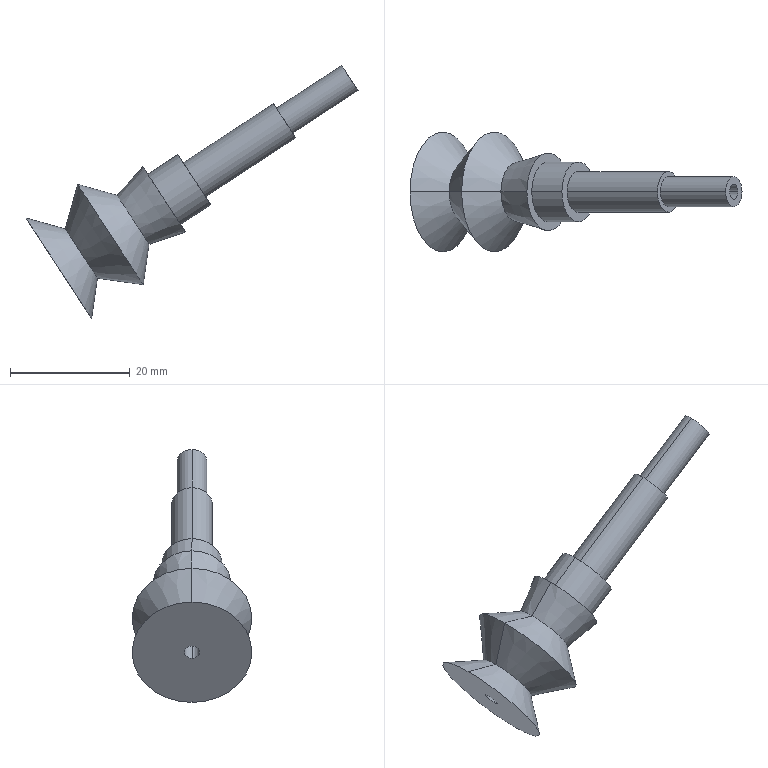Component | SolidWorks | NewSuctionCupGroup-1_SuctionCup1-1 | 1 solid | 21 faces | box 55.39 x 20 x 42.19 mm | volume 4409 mm3 | cylinder 8 | cone 8 | plane 5 | commonest cylinder face diameters 2.5 x2 10 x2 6.8 x2 5 x2
build123d program:
from build123d import *

# Parameters (mm, degrees)
SKETCH2_R          = 1.25
CUT_EXTRUDE1_DEPTH = 60.699


with BuildPart() as part:
    # Sketch1 → Revolve1 (revolve)
    with BuildSketch(Plane.XY, mode=Mode.PRIVATE) as revolve1_sk:
        Polygon((0, 0), (2.5, 0), (2.5, -13), (3.4, -13), (3.4, -31), (5, -31), (5, -37), (6.489, -37), (4.895, -43.22), (10, -47.704), (4.895, -53.516), (10, -58), (0, -58), align=None)
    revolve(revolve1_sk.sketch.rotate(Axis((0, 0, 0), (0, -1, 0)), 90), axis=Axis((0, 0, 0), (0, -1, 0)))

    # Sketch2 → Cut-Extrude1 (cut, through all)
    with BuildSketch(Plane.XZ.offset(58)):
        with Locations(Location((0, 0, 0), (0, 0, 270))):
            Circle(SKETCH2_R)
    extrude(amount=-CUT_EXTRUDE1_DEPTH, mode=Mode.SUBTRACT)


solid = part.part

# Placed as in the assembly
solid = solid.moved(Location((-65.517, -100.454, -13.641), (175.111, 33.07, -87.328)))
STEP:
#1=CARTESIAN_POINT('',(-2.606,-3.955,-0.4958));
#2=VERTEX_POINT('',#1);
#3=CARTESIAN_POINT('',(-2.552,-3.955,-0.5782));
#4=VERTEX_POINT('',#3);
#5=CARTESIAN_POINT('',(-2.579,-3.955,-0.537));
#6=DIRECTION('',(-0.8371,0.,-0.5471));
#7=DIRECTION('',(0.5471,0.,-0.8371));
#8=AXIS2_PLACEMENT_3D('',#5,#6,#7);
#9=CIRCLE('',#8,0.04921);
#10=EDGE_CURVE('',#2,#4,#9,.T.);
#11=ORIENTED_EDGE('',*,*,#10,.F.);
#12=CARTESIAN_POINT('',(-4.518,-3.955,-1.745));
#13=VERTEX_POINT('',#12);
#14=CARTESIAN_POINT('',(-2.606,-3.955,-0.4958));
#15=DIRECTION('',(-0.8371,0.,-0.5471));
#16=VECTOR('',#15,39.37);
#17=LINE('',#14,#16);
#18=EDGE_CURVE('',#2,#13,#17,.T.);
#19=ORIENTED_EDGE('',*,*,#18,.T.);
#20=CARTESIAN_POINT('',(-4.464,-3.955,-1.827));
#21=VERTEX_POINT('',#20);
#22=CARTESIAN_POINT('',(-4.491,-3.955,-1.786));
#23=DIRECTION('',(-0.8371,0.,-0.5471));
#24=DIRECTION('',(0.5471,0.,-0.8371));
#25=AXIS2_PLACEMENT_3D('',#22,#23,#24);
#26=CIRCLE('',#25,0.04921);
#27=EDGE_CURVE('',#13,#21,#26,.T.);
#28=ORIENTED_EDGE('',*,*,#27,.T.);
#29=CARTESIAN_POINT('',(-2.552,-3.955,-0.5782));
#30=DIRECTION('',(-0.8371,0.,-0.5471));
#31=VECTOR('',#30,39.37);
#32=LINE('',#29,#31);
#33=EDGE_CURVE('',#4,#21,#32,.T.);
#34=ORIENTED_EDGE('',*,*,#33,.F.);
#35=EDGE_LOOP('',(#11,#19,#28,#34));
#36=FACE_OUTER_BOUND('',#35,.T.);
#37=CARTESIAN_POINT('',(-2.579,-3.955,-0.537));
#38=DIRECTION('',(-0.8371,0.,-0.5471));
#39=DIRECTION('',(0.5471,0.,-0.8371));
#40=AXIS2_PLACEMENT_3D('',#37,#38,#39);
#41=CYLINDRICAL_SURFACE('',#40,0.04921);
#42=ADVANCED_FACE('',(#36),#41,.F.);
#43=CARTESIAN_POINT('',(-4.449,-3.955,-1.528));
#44=VERTEX_POINT('',#43);
#45=CARTESIAN_POINT('',(-4.238,-3.955,-1.851));
#46=VERTEX_POINT('',#45);
#47=CARTESIAN_POINT('',(-4.343,-3.955,-1.69));
#48=DIRECTION('',(0.8371,-0.,0.5471));
#49=DIRECTION('',(-0.5471,0.,0.8371));
#50=AXIS2_PLACEMENT_3D('',#47,#48,#49);
#51=CIRCLE('',#50,0.1927);
#52=EDGE_CURVE('',#44,#46,#51,.T.);
#53=ORIENTED_EDGE('',*,*,#52,.F.);
#54=CARTESIAN_POINT('',(-4.706,-3.955,-1.457));
#55=VERTEX_POINT('',#54);
#56=CARTESIAN_POINT('',(-4.706,-3.955,-1.457));
#57=DIRECTION('',(-0.9634,0.,0.2679));
#58=VECTOR('',#57,39.37);
#59=LINE('',#56,#58);
#60=EDGE_CURVE('',#44,#55,#59,.T.);
#61=ORIENTED_EDGE('',*,*,#60,.T.);
#62=CARTESIAN_POINT('',(-4.276,-3.955,-2.116));
#63=VERTEX_POINT('',#62);
#64=CARTESIAN_POINT('',(-4.491,-3.955,-1.786));
#65=DIRECTION('',(0.8371,-0.,0.5471));
#66=DIRECTION('',(-0.5471,0.,0.8371));
#67=AXIS2_PLACEMENT_3D('',#64,#65,#66);
#68=CIRCLE('',#67,0.3937);
#69=EDGE_CURVE('',#55,#63,#68,.T.);
#70=ORIENTED_EDGE('',*,*,#69,.T.);
#71=CARTESIAN_POINT('',(-4.276,-3.955,-2.116));
#72=DIRECTION('',(-0.1414,-0.,-0.99));
#73=VECTOR('',#72,39.37);
#74=LINE('',#71,#73);
#75=EDGE_CURVE('',#46,#63,#74,.T.);
#76=ORIENTED_EDGE('',*,*,#75,.F.);
#77=EDGE_LOOP('',(#53,#61,#70,#76));
#78=FACE_OUTER_BOUND('',#77,.T.);
#79=CARTESIAN_POINT('',(-4.491,-3.955,-1.786));
#80=DIRECTION('',(-0.8371,0.,-0.5471));
#81=DIRECTION('',(0.5471,-0.,-0.8371));
#82=AXIS2_PLACEMENT_3D('',#79,#80,#81);
#83=CONICAL_SURFACE('',#82,0.3937,0.8501);
#84=ADVANCED_FACE('',(#78),#83,.T.);
#85=ORIENTED_EDGE('',*,*,#52,.T.);
#86=CARTESIAN_POINT('',(-3.936,-3.955,-1.894));
#87=VERTEX_POINT('',#86);
#88=CARTESIAN_POINT('',(-4.238,-3.955,-1.851));
#89=DIRECTION('',(0.99,-0.,-0.1414));
#90=VECTOR('',#89,39.37);
#91=LINE('',#88,#90);
#92=EDGE_CURVE('',#46,#87,#91,.T.);
#93=ORIENTED_EDGE('',*,*,#92,.T.);
#94=CARTESIAN_POINT('',(-4.367,-3.955,-1.235));
#95=VERTEX_POINT('',#94);
#96=CARTESIAN_POINT('',(-4.152,-3.955,-1.564));
#97=DIRECTION('',(0.8371,-0.,0.5471));
#98=DIRECTION('',(-0.5471,0.,0.8371));
#99=AXIS2_PLACEMENT_3D('',#96,#97,#98);
#100=CIRCLE('',#99,0.3937);
#101=EDGE_CURVE('',#95,#87,#100,.T.);
#102=ORIENTED_EDGE('',*,*,#101,.F.);
#103=CARTESIAN_POINT('',(-4.449,-3.955,-1.528));
#104=DIRECTION('',(0.2679,0.,0.9634));
#105=VECTOR('',#104,39.37);
#106=LINE('',#103,#105);
#107=EDGE_CURVE('',#44,#95,#106,.T.);
#108=ORIENTED_EDGE('',*,*,#107,.F.);
#109=EDGE_LOOP('',(#85,#93,#102,#108));
#110=FACE_OUTER_BOUND('',#109,.T.);
#111=CARTESIAN_POINT('',(-4.343,-3.955,-1.69));
#112=DIRECTION('',(0.8371,-0.,0.5471));
#113=DIRECTION('',(-0.5471,0.,0.8371));
#114=AXIS2_PLACEMENT_3D('',#111,#112,#113);
#115=CONICAL_SURFACE('',#114,0.1927,0.7207);
#116=ADVANCED_FACE('',(#110),#115,.T.);
#117=CARTESIAN_POINT('',(-4.109,-3.955,-1.307));
#118=VERTEX_POINT('',#117);
#119=CARTESIAN_POINT('',(-3.898,-3.955,-1.629));
#120=VERTEX_POINT('',#119);
#121=CARTESIAN_POINT('',(-4.004,-3.955,-1.468));
#122=DIRECTION('',(0.8371,-0.,0.5471));
#123=DIRECTION('',(-0.5471,0.,0.8371));
#124=AXIS2_PLACEMENT_3D('',#121,#122,#123);
#125=CIRCLE('',#124,0.1927);
#126=EDGE_CURVE('',#118,#120,#125,.T.);
#127=ORIENTED_EDGE('',*,*,#126,.F.);
#128=CARTESIAN_POINT('',(-4.367,-3.955,-1.235));
#129=DIRECTION('',(-0.9634,0.,0.2679));
#130=VECTOR('',#129,39.37);
#131=LINE('',#128,#130);
#132=EDGE_CURVE('',#118,#95,#131,.T.);
#133=ORIENTED_EDGE('',*,*,#132,.T.);
#134=ORIENTED_EDGE('',*,*,#101,.T.);
#135=CARTESIAN_POINT('',(-3.936,-3.955,-1.894));
#136=DIRECTION('',(-0.1414,-0.,-0.99));
#137=VECTOR('',#136,39.37);
#138=LINE('',#135,#137);
#139=EDGE_CURVE('',#120,#87,#138,.T.);
#140=ORIENTED_EDGE('',*,*,#139,.F.);
#141=EDGE_LOOP('',(#127,#133,#134,#140));
#142=FACE_OUTER_BOUND('',#141,.T.);
#143=CARTESIAN_POINT('',(-4.152,-3.955,-1.564));
#144=DIRECTION('',(-0.8371,0.,-0.5471));
#145=DIRECTION('',(0.5471,-0.,-0.8371));
#146=AXIS2_PLACEMENT_3D('',#143,#144,#145);
#147=CONICAL_SURFACE('',#146,0.3937,0.8501);
#148=ADVANCED_FACE('',(#142),#147,.T.);
#149=ORIENTED_EDGE('',*,*,#126,.T.);
#150=CARTESIAN_POINT('',(-3.659,-3.955,-1.548));
#151=VERTEX_POINT('',#150);
#152=CARTESIAN_POINT('',(-3.898,-3.955,-1.629));
#153=DIRECTION('',(0.9467,-0.,0.3221));
#154=VECTOR('',#153,39.37);
#155=LINE('',#152,#154);
#156=EDGE_CURVE('',#120,#151,#155,.T.);
#157=ORIENTED_EDGE('',*,*,#156,.T.);
#158=CARTESIAN_POINT('',(-3.939,-3.955,-1.12));
#159=VERTEX_POINT('',#158);
#160=CARTESIAN_POINT('',(-3.799,-3.955,-1.334));
#161=DIRECTION('',(0.8371,-0.,0.5471));
#162=DIRECTION('',(-0.5471,0.,0.8371));
#163=AXIS2_PLACEMENT_3D('',#160,#161,#162);
#164=CIRCLE('',#163,0.2555);
#165=EDGE_CURVE('',#159,#151,#164,.T.);
#166=ORIENTED_EDGE('',*,*,#165,.F.);
#167=CARTESIAN_POINT('',(-4.109,-3.955,-1.307));
#168=DIRECTION('',(0.6751,-0.,0.7377));
#169=VECTOR('',#168,39.37);
#170=LINE('',#167,#169);
#171=EDGE_CURVE('',#118,#159,#170,.T.);
#172=ORIENTED_EDGE('',*,*,#171,.F.);
#173=EDGE_LOOP('',(#149,#157,#166,#172));
#174=FACE_OUTER_BOUND('',#173,.T.);
#175=CARTESIAN_POINT('',(-4.004,-3.955,-1.468));
#176=DIRECTION('',(0.8371,-0.,0.5471));
#177=DIRECTION('',(-0.5471,0.,0.8371));
#178=AXIS2_PLACEMENT_3D('',#175,#176,#177);
#179=CONICAL_SURFACE('',#178,0.1927,0.2509);
#180=ADVANCED_FACE('',(#174),#179,.T.);
#181=CARTESIAN_POINT('',(-3.906,-3.955,-1.169));
#182=VERTEX_POINT('',#181);
#183=CARTESIAN_POINT('',(-3.691,-3.955,-1.499));
#184=VERTEX_POINT('',#183);
#185=CARTESIAN_POINT('',(-3.799,-3.955,-1.334));
#186=DIRECTION('',(0.8371,-0.,0.5471));
#187=DIRECTION('',(-0.5471,0.,0.8371));
#188=AXIS2_PLACEMENT_3D('',#185,#186,#187);
#189=CIRCLE('',#188,0.1969);
#190=EDGE_CURVE('',#182,#184,#189,.T.);
#191=ORIENTED_EDGE('',*,*,#190,.T.);
#192=CARTESIAN_POINT('',(-3.493,-3.955,-1.369));
#193=VERTEX_POINT('',#192);
#194=CARTESIAN_POINT('',(-2.472,-3.955,-0.7018));
#195=DIRECTION('',(0.8371,-0.,0.5471));
#196=VECTOR('',#195,39.37);
#197=LINE('',#194,#196);
#198=EDGE_CURVE('',#184,#193,#197,.T.);
#199=ORIENTED_EDGE('',*,*,#198,.T.);
#200=CARTESIAN_POINT('',(-3.709,-3.955,-1.04));
#201=VERTEX_POINT('',#200);
#202=CARTESIAN_POINT('',(-3.601,-3.955,-1.205));
#203=DIRECTION('',(0.8371,-0.,0.5471));
#204=DIRECTION('',(-0.5471,0.,0.8371));
#205=AXIS2_PLACEMENT_3D('',#202,#203,#204);
#206=CIRCLE('',#205,0.1969);
#207=EDGE_CURVE('',#201,#193,#206,.T.);
#208=ORIENTED_EDGE('',*,*,#207,.F.);
#209=CARTESIAN_POINT('',(-2.687,-3.955,-0.3723));
#210=DIRECTION('',(0.8371,-0.,0.5471));
#211=VECTOR('',#210,39.37);
#212=LINE('',#209,#211);
#213=EDGE_CURVE('',#182,#201,#212,.T.);
#214=ORIENTED_EDGE('',*,*,#213,.F.);
#215=EDGE_LOOP('',(#191,#199,#208,#214));
#216=FACE_OUTER_BOUND('',#215,.T.);
#217=CARTESIAN_POINT('',(-2.579,-3.955,-0.537));
#218=DIRECTION('',(0.8371,-0.,0.5471));
#219=DIRECTION('',(-0.5471,0.,0.8371));
#220=AXIS2_PLACEMENT_3D('',#217,#218,#219);
#221=CYLINDRICAL_SURFACE('',#220,0.1969);
#222=ADVANCED_FACE('',(#216),#221,.T.);
#223=CARTESIAN_POINT('',(-3.674,-3.955,-1.093));
#224=VERTEX_POINT('',#223);
#225=CARTESIAN_POINT('',(-3.528,-3.955,-1.317));
#226=VERTEX_POINT('',#225);
#227=CARTESIAN_POINT('',(-3.601,-3.955,-1.205));
#228=DIRECTION('',(0.8371,-0.,0.5471));
#229=DIRECTION('',(-0.5471,0.,0.8371));
#230=AXIS2_PLACEMENT_3D('',#227,#228,#229);
#231=CIRCLE('',#230,0.1339);
#232=EDGE_CURVE('',#224,#226,#231,.T.);
#233=ORIENTED_EDGE('',*,*,#232,.T.);
#234=CARTESIAN_POINT('',(-2.935,-3.955,-0.9291));
#235=VERTEX_POINT('',#234);
#236=CARTESIAN_POINT('',(-2.506,-3.955,-0.6491));
#237=DIRECTION('',(0.8371,-0.,0.5471));
#238=VECTOR('',#237,39.37);
#239=LINE('',#236,#238);
#240=EDGE_CURVE('',#226,#235,#239,.T.);
#241=ORIENTED_EDGE('',*,*,#240,.T.);
#242=CARTESIAN_POINT('',(-3.081,-3.955,-0.705));
#243=VERTEX_POINT('',#242);
#244=CARTESIAN_POINT('',(-3.008,-3.955,-0.817));
#245=DIRECTION('',(0.8371,-0.,0.5471));
#246=DIRECTION('',(-0.5471,0.,0.8371));
#247=AXIS2_PLACEMENT_3D('',#244,#245,#246);
#248=CIRCLE('',#247,0.1339);
#249=EDGE_CURVE('',#243,#235,#248,.T.);
#250=ORIENTED_EDGE('',*,*,#249,.F.);
#251=CARTESIAN_POINT('',(-2.653,-3.955,-0.425));
#252=DIRECTION('',(0.8371,-0.,0.5471));
#253=VECTOR('',#252,39.37);
#254=LINE('',#251,#253);
#255=EDGE_CURVE('',#224,#243,#254,.T.);
#256=ORIENTED_EDGE('',*,*,#255,.F.);
#257=EDGE_LOOP('',(#233,#241,#250,#256));
#258=FACE_OUTER_BOUND('',#257,.T.);
#259=CARTESIAN_POINT('',(-2.579,-3.955,-0.537));
#260=DIRECTION('',(0.8371,-0.,0.5471));
#261=DIRECTION('',(-0.5471,0.,0.8371));
#262=AXIS2_PLACEMENT_3D('',#259,#260,#261);
#263=CYLINDRICAL_SURFACE('',#262,0.1339);
#264=ADVANCED_FACE('',(#258),#263,.T.);
#265=CARTESIAN_POINT('',(-3.062,-3.955,-0.7346));
#266=VERTEX_POINT('',#265);
#267=CARTESIAN_POINT('',(-2.954,-3.955,-0.8994));
#268=VERTEX_POINT('',#267);
#269=CARTESIAN_POINT('',(-3.008,-3.955,-0.817));
#270=DIRECTION('',(0.8371,-0.,0.5471));
#271=DIRECTION('',(-0.5471,0.,0.8371));
#272=AXIS2_PLACEMENT_3D('',#269,#270,#271);
#273=CIRCLE('',#272,0.09843);
#274=EDGE_CURVE('',#266,#268,#273,.T.);
#275=ORIENTED_EDGE('',*,*,#274,.T.);
#276=CARTESIAN_POINT('',(-2.526,-3.955,-0.6194));
#277=VERTEX_POINT('',#276);
#278=CARTESIAN_POINT('',(-2.526,-3.955,-0.6194));
#279=DIRECTION('',(0.8371,-0.,0.5471));
#280=VECTOR('',#279,39.37);
#281=LINE('',#278,#280);
#282=EDGE_CURVE('',#268,#277,#281,.T.);
#283=ORIENTED_EDGE('',*,*,#282,.T.);
#284=CARTESIAN_POINT('',(-2.633,-3.955,-0.4546));
#285=VERTEX_POINT('',#284);
#286=CARTESIAN_POINT('',(-2.579,-3.955,-0.537));
#287=DIRECTION('',(0.8371,-0.,0.5471));
#288=DIRECTION('',(-0.5471,0.,0.8371));
#289=AXIS2_PLACEMENT_3D('',#286,#287,#288);
#290=CIRCLE('',#289,0.09843);
#291=EDGE_CURVE('',#285,#277,#290,.T.);
#292=ORIENTED_EDGE('',*,*,#291,.F.);
#293=CARTESIAN_POINT('',(-2.633,-3.955,-0.4546));
#294=DIRECTION('',(0.8371,-0.,0.5471));
#295=VECTOR('',#294,39.37);
#296=LINE('',#293,#295);
#297=EDGE_CURVE('',#266,#285,#296,.T.);
#298=ORIENTED_EDGE('',*,*,#297,.F.);
#299=EDGE_LOOP('',(#275,#283,#292,#298));
#300=FACE_OUTER_BOUND('',#299,.T.);
#301=CARTESIAN_POINT('',(-2.579,-3.955,-0.537));
#302=DIRECTION('',(0.8371,-0.,0.5471));
#303=DIRECTION('',(-0.5471,0.,0.8371));
#304=AXIS2_PLACEMENT_3D('',#301,#302,#303);
#305=CYLINDRICAL_SURFACE('',#304,0.09843);
#306=ADVANCED_FACE('',(#300),#305,.T.);
#307=CARTESIAN_POINT('',(-2.579,-3.955,-0.537));
#308=DIRECTION('',(-0.8371,0.,-0.5471));
#309=DIRECTION('',(0.5471,0.,-0.8371));
#310=AXIS2_PLACEMENT_3D('',#307,#308,#309);
#311=CIRCLE('',#310,0.04921);
#312=EDGE_CURVE('',#4,#2,#311,.T.);
#313=ORIENTED_EDGE('',*,*,#312,.T.);
#314=ORIENTED_EDGE('',*,*,#10,.T.);
#315=EDGE_LOOP('',(#313,#314));
#316=FACE_BOUND('',#315,.T.);
#317=ORIENTED_EDGE('',*,*,#291,.T.);
#318=CARTESIAN_POINT('',(-2.579,-3.955,-0.537));
#319=DIRECTION('',(0.8371,-0.,0.5471));
#320=DIRECTION('',(-0.5471,0.,0.8371));
#321=AXIS2_PLACEMENT_3D('',#318,#319,#320);
#322=CIRCLE('',#321,0.09843);
#323=EDGE_CURVE('',#277,#285,#322,.T.);
#324=ORIENTED_EDGE('',*,*,#323,.T.);
#325=EDGE_LOOP('',(#317,#324));
#326=FACE_OUTER_BOUND('',#325,.T.);
#327=CARTESIAN_POINT('',(-2.579,-3.955,-0.537));
#328=DIRECTION('',(-0.8371,0.,-0.5471));
#329=DIRECTION('',(0.5471,-0.,-0.8371));
#330=AXIS2_PLACEMENT_3D('',#327,#328,#329);
#331=PLANE('',#330);
#332=ADVANCED_FACE('',(#316,#326),#331,.F.);
#333=ORIENTED_EDGE('',*,*,#282,.F.);
#334=CARTESIAN_POINT('',(-3.008,-3.955,-0.817));
#335=DIRECTION('',(0.8371,-0.,0.5471));
#336=DIRECTION('',(-0.5471,0.,0.8371));
#337=AXIS2_PLACEMENT_3D('',#334,#335,#336);
#338=CIRCLE('',#337,0.09843);
#339=EDGE_CURVE('',#268,#266,#338,.T.);
#340=ORIENTED_EDGE('',*,*,#339,.T.);
#341=ORIENTED_EDGE('',*,*,#297,.T.);
#342=ORIENTED_EDGE('',*,*,#323,.F.);
#343=EDGE_LOOP('',(#333,#340,#341,#342));
#344=FACE_OUTER_BOUND('',#343,.T.);
#345=CARTESIAN_POINT('',(-2.579,-3.955,-0.537));
#346=DIRECTION('',(0.8371,-0.,0.5471));
#347=DIRECTION('',(-0.5471,0.,0.8371));
#348=AXIS2_PLACEMENT_3D('',#345,#346,#347);
#349=CYLINDRICAL_SURFACE('',#348,0.09843);
#350=ADVANCED_FACE('',(#344),#349,.T.);
#351=ORIENTED_EDGE('',*,*,#274,.F.);
#352=ORIENTED_EDGE('',*,*,#339,.F.);
#353=EDGE_LOOP('',(#351,#352));
#354=FACE_BOUND('',#353,.T.);
#355=ORIENTED_EDGE('',*,*,#249,.T.);
#356=CARTESIAN_POINT('',(-3.008,-3.955,-0.817));
#357=DIRECTION('',(0.8371,-0.,0.5471));
#358=DIRECTION('',(-0.5471,0.,0.8371));
#359=AXIS2_PLACEMENT_3D('',#356,#357,#358);
#360=CIRCLE('',#359,0.1339);
#361=EDGE_CURVE('',#235,#243,#360,.T.);
#362=ORIENTED_EDGE('',*,*,#361,.T.);
#363=EDGE_LOOP('',(#355,#362));
#364=FACE_OUTER_BOUND('',#363,.T.);
#365=CARTESIAN_POINT('',(-3.008,-4.053,-0.817));
#366=DIRECTION('',(-0.8371,0.,-0.5471));
#367=DIRECTION('',(0.5471,-0.,-0.8371));
#368=AXIS2_PLACEMENT_3D('',#365,#366,#367);
#369=PLANE('',#368);
#370=ADVANCED_FACE('',(#354,#364),#369,.F.);
#371=ORIENTED_EDGE('',*,*,#240,.F.);
#372=CARTESIAN_POINT('',(-3.601,-3.955,-1.205));
#373=DIRECTION('',(0.8371,-0.,0.5471));
#374=DIRECTION('',(-0.5471,0.,0.8371));
#375=AXIS2_PLACEMENT_3D('',#372,#373,#374);
#376=CIRCLE('',#375,0.1339);
#377=EDGE_CURVE('',#226,#224,#376,.T.);
#378=ORIENTED_EDGE('',*,*,#377,.T.);
#379=ORIENTED_EDGE('',*,*,#255,.T.);
#380=ORIENTED_EDGE('',*,*,#361,.F.);
#381=EDGE_LOOP('',(#371,#378,#379,#380));
#382=FACE_OUTER_BOUND('',#381,.T.);
#383=CARTESIAN_POINT('',(-2.579,-3.955,-0.537));
#384=DIRECTION('',(0.8371,-0.,0.5471));
#385=DIRECTION('',(-0.5471,0.,0.8371));
#386=AXIS2_PLACEMENT_3D('',#383,#384,#385);
#387=CYLINDRICAL_SURFACE('',#386,0.1339);
#388=ADVANCED_FACE('',(#382),#387,.T.);
#389=ORIENTED_EDGE('',*,*,#232,.F.);
#390=ORIENTED_EDGE('',*,*,#377,.F.);
#391=EDGE_LOOP('',(#389,#390));
#392=FACE_BOUND('',#391,.T.);
#393=ORIENTED_EDGE('',*,*,#207,.T.);
#394=CARTESIAN_POINT('',(-3.601,-3.955,-1.205));
#395=DIRECTION('',(0.8371,-0.,0.5471));
#396=DIRECTION('',(-0.5471,0.,0.8371));
#397=AXIS2_PLACEMENT_3D('',#394,#395,#396);
#398=CIRCLE('',#397,0.1969);
#399=EDGE_CURVE('',#193,#201,#398,.T.);
#400=ORIENTED_EDGE('',*,*,#399,.T.);
#401=EDGE_LOOP('',(#393,#400));
#402=FACE_OUTER_BOUND('',#401,.T.);
#403=CARTESIAN_POINT('',(-3.601,-4.089,-1.205));
#404=DIRECTION('',(-0.8371,0.,-0.5471));
#405=DIRECTION('',(0.5471,-0.,-0.8371));
#406=AXIS2_PLACEMENT_3D('',#403,#404,#405);
#407=PLANE('',#406);
#408=ADVANCED_FACE('',(#392,#402),#407,.F.);
#409=ORIENTED_EDGE('',*,*,#198,.F.);
#410=CARTESIAN_POINT('',(-3.799,-3.955,-1.334));
#411=DIRECTION('',(0.8371,-0.,0.5471));
#412=DIRECTION('',(-0.5471,0.,0.8371));
#413=AXIS2_PLACEMENT_3D('',#410,#411,#412);
#414=CIRCLE('',#413,0.1969);
#415=EDGE_CURVE('',#184,#182,#414,.T.);
#416=ORIENTED_EDGE('',*,*,#415,.T.);
#417=ORIENTED_EDGE('',*,*,#213,.T.);
#418=ORIENTED_EDGE('',*,*,#399,.F.);
#419=EDGE_LOOP('',(#409,#416,#417,#418));
#420=FACE_OUTER_BOUND('',#419,.T.);
#421=CARTESIAN_POINT('',(-2.579,-3.955,-0.537));
#422=DIRECTION('',(0.8371,-0.,0.5471));
#423=DIRECTION('',(-0.5471,0.,0.8371));
#424=AXIS2_PLACEMENT_3D('',#421,#422,#423);
#425=CYLINDRICAL_SURFACE('',#424,0.1969);
#426=ADVANCED_FACE('',(#420),#425,.T.);
#427=ORIENTED_EDGE('',*,*,#190,.F.);
#428=ORIENTED_EDGE('',*,*,#415,.F.);
#429=EDGE_LOOP('',(#427,#428));
#430=FACE_BOUND('',#429,.T.);
#431=ORIENTED_EDGE('',*,*,#165,.T.);
#432=CARTESIAN_POINT('',(-3.799,-3.955,-1.334));
#433=DIRECTION('',(0.8371,-0.,0.5471));
#434=DIRECTION('',(-0.5471,0.,0.8371));
#435=AXIS2_PLACEMENT_3D('',#432,#433,#434);
#436=CIRCLE('',#435,0.2555);
#437=EDGE_CURVE('',#151,#159,#436,.T.);
#438=ORIENTED_EDGE('',*,*,#437,.T.);
#439=EDGE_LOOP('',(#431,#438));
#440=FACE_OUTER_BOUND('',#439,.T.);
#441=CARTESIAN_POINT('',(-3.799,-4.152,-1.334));
#442=DIRECTION('',(-0.8371,0.,-0.5471));
#443=DIRECTION('',(0.5471,-0.,-0.8371));
#444=AXIS2_PLACEMENT_3D('',#441,#442,#443);
#445=PLANE('',#444);
#446=ADVANCED_FACE('',(#430,#440),#445,.F.);
#447=ORIENTED_EDGE('',*,*,#156,.F.);
#448=CARTESIAN_POINT('',(-4.004,-3.955,-1.468));
#449=DIRECTION('',(0.8371,-0.,0.5471));
#450=DIRECTION('',(-0.5471,0.,0.8371));
#451=AXIS2_PLACEMENT_3D('',#448,#449,#450);
#452=CIRCLE('',#451,0.1927);
#453=EDGE_CURVE('',#120,#118,#452,.T.);
#454=ORIENTED_EDGE('',*,*,#453,.T.);
#455=ORIENTED_EDGE('',*,*,#171,.T.);
#456=ORIENTED_EDGE('',*,*,#437,.F.);
#457=EDGE_LOOP('',(#447,#454,#455,#456));
#458=FACE_OUTER_BOUND('',#457,.T.);
#459=CARTESIAN_POINT('',(-4.004,-3.955,-1.468));
#460=DIRECTION('',(0.8371,-0.,0.5471));
#461=DIRECTION('',(-0.5471,0.,0.8371));
#462=AXIS2_PLACEMENT_3D('',#459,#460,#461);
#463=CONICAL_SURFACE('',#462,0.1927,0.2509);
#464=ADVANCED_FACE('',(#458),#463,.T.);
#465=ORIENTED_EDGE('',*,*,#132,.F.);
#466=ORIENTED_EDGE('',*,*,#453,.F.);
#467=ORIENTED_EDGE('',*,*,#139,.T.);
#468=CARTESIAN_POINT('',(-4.152,-3.955,-1.564));
#469=DIRECTION('',(0.8371,-0.,0.5471));
#470=DIRECTION('',(-0.5471,0.,0.8371));
#471=AXIS2_PLACEMENT_3D('',#468,#469,#470);
#472=CIRCLE('',#471,0.3937);
#473=EDGE_CURVE('',#87,#95,#472,.T.);
#474=ORIENTED_EDGE('',*,*,#473,.T.);
#475=EDGE_LOOP('',(#465,#466,#467,#474));
#476=FACE_OUTER_BOUND('',#475,.T.);
#477=CARTESIAN_POINT('',(-4.152,-3.955,-1.564));
#478=DIRECTION('',(-0.8371,0.,-0.5471));
#479=DIRECTION('',(0.5471,-0.,-0.8371));
#480=AXIS2_PLACEMENT_3D('',#477,#478,#479);
#481=CONICAL_SURFACE('',#480,0.3937,0.8501);
#482=ADVANCED_FACE('',(#476),#481,.T.);
#483=ORIENTED_EDGE('',*,*,#92,.F.);
#484=CARTESIAN_POINT('',(-4.343,-3.955,-1.69));
#485=DIRECTION('',(0.8371,-0.,0.5471));
#486=DIRECTION('',(-0.5471,0.,0.8371));
#487=AXIS2_PLACEMENT_3D('',#484,#485,#486);
#488=CIRCLE('',#487,0.1927);
#489=EDGE_CURVE('',#46,#44,#488,.T.);
#490=ORIENTED_EDGE('',*,*,#489,.T.);
#491=ORIENTED_EDGE('',*,*,#107,.T.);
#492=ORIENTED_EDGE('',*,*,#473,.F.);
#493=EDGE_LOOP('',(#483,#490,#491,#492));
#494=FACE_OUTER_BOUND('',#493,.T.);
#495=CARTESIAN_POINT('',(-4.343,-3.955,-1.69));
#496=DIRECTION('',(0.8371,-0.,0.5471));
#497=DIRECTION('',(-0.5471,0.,0.8371));
#498=AXIS2_PLACEMENT_3D('',#495,#496,#497);
#499=CONICAL_SURFACE('',#498,0.1927,0.7207);
#500=ADVANCED_FACE('',(#494),#499,.T.);
#501=ORIENTED_EDGE('',*,*,#60,.F.);
#502=ORIENTED_EDGE('',*,*,#489,.F.);
#503=ORIENTED_EDGE('',*,*,#75,.T.);
#504=CARTESIAN_POINT('',(-4.491,-3.955,-1.786));
#505=DIRECTION('',(0.8371,-0.,0.5471));
#506=DIRECTION('',(-0.5471,0.,0.8371));
#507=AXIS2_PLACEMENT_3D('',#504,#505,#506);
#508=CIRCLE('',#507,0.3937);
#509=EDGE_CURVE('',#63,#55,#508,.T.);
#510=ORIENTED_EDGE('',*,*,#509,.T.);
#511=EDGE_LOOP('',(#501,#502,#503,#510));
#512=FACE_OUTER_BOUND('',#511,.T.);
#513=CARTESIAN_POINT('',(-4.491,-3.955,-1.786));
#514=DIRECTION('',(-0.8371,0.,-0.5471));
#515=DIRECTION('',(0.5471,-0.,-0.8371));
#516=AXIS2_PLACEMENT_3D('',#513,#514,#515);
#517=CONICAL_SURFACE('',#516,0.3937,0.8501);
#518=ADVANCED_FACE('',(#512),#517,.T.);
#519=CARTESIAN_POINT('',(-4.491,-3.955,-1.786));
#520=DIRECTION('',(-0.8371,0.,-0.5471));
#521=DIRECTION('',(0.5471,0.,-0.8371));
#522=AXIS2_PLACEMENT_3D('',#519,#520,#521);
#523=CIRCLE('',#522,0.04921);
#524=EDGE_CURVE('',#21,#13,#523,.T.);
#525=ORIENTED_EDGE('',*,*,#524,.F.);
#526=ORIENTED_EDGE('',*,*,#27,.F.);
#527=EDGE_LOOP('',(#525,#526));
#528=FACE_BOUND('',#527,.T.);
#529=ORIENTED_EDGE('',*,*,#509,.F.);
#530=ORIENTED_EDGE('',*,*,#69,.F.);
#531=EDGE_LOOP('',(#529,#530));
#532=FACE_OUTER_BOUND('',#531,.T.);
#533=CARTESIAN_POINT('',(-4.491,-4.349,-1.786));
#534=DIRECTION('',(0.8371,-0.,0.5471));
#535=DIRECTION('',(-0.5471,0.,0.8371));
#536=AXIS2_PLACEMENT_3D('',#533,#534,#535);
#537=PLANE('',#536);
#538=ADVANCED_FACE('',(#528,#532),#537,.F.);
#539=ORIENTED_EDGE('',*,*,#18,.F.);
#540=ORIENTED_EDGE('',*,*,#312,.F.);
#541=ORIENTED_EDGE('',*,*,#33,.T.);
#542=ORIENTED_EDGE('',*,*,#524,.T.);
#543=EDGE_LOOP('',(#539,#540,#541,#542));
#544=FACE_OUTER_BOUND('',#543,.T.);
#545=CARTESIAN_POINT('',(-2.579,-3.955,-0.537));
#546=DIRECTION('',(-0.8371,0.,-0.5471));
#547=DIRECTION('',(0.5471,0.,-0.8371));
#548=AXIS2_PLACEMENT_3D('',#545,#546,#547);
#549=CYLINDRICAL_SURFACE('',#548,0.04921);
#550=ADVANCED_FACE('',(#544),#549,.F.);
#551=CLOSED_SHELL('',(#42,#84,#116,#148,#180,#222,#264,#306,#332,#350,#370,#388,#408,#426,#446,#464,#482,#500,#518,#538,#550));
#552=MANIFOLD_SOLID_BREP('',#551);
#553=CARTESIAN_POINT('',(0.,0.,0.));
#554=DIRECTION('',(0.,0.,1.));
#555=DIRECTION('',(1.,0.,0.));
#556=AXIS2_PLACEMENT_3D('',#553,#554,#555);
#557=(LENGTH_UNIT()NAMED_UNIT(*)SI_UNIT($,.METRE.));
#558=LENGTH_MEASURE_WITH_UNIT(LENGTH_MEASURE(0.0254),#557);
#559=DIMENSIONAL_EXPONENTS(1.,0.,0.,0.,0.,0.,0.);
#560=(CONVERSION_BASED_UNIT('',#558)LENGTH_UNIT()NAMED_UNIT(#559));
#561=UNCERTAINTY_MEASURE_WITH_UNIT(LENGTH_MEASURE(0.00001),#560,'','');
#562=(NAMED_UNIT(*)PLANE_ANGLE_UNIT()SI_UNIT($,.RADIAN.));
#563=(NAMED_UNIT(*)SI_UNIT($,.STERADIAN.)SOLID_ANGLE_UNIT());
#564=(GEOMETRIC_REPRESENTATION_CONTEXT(3)GLOBAL_UNCERTAINTY_ASSIGNED_CONTEXT((#561))GLOBAL_UNIT_ASSIGNED_CONTEXT((#560,#562,#563))REPRESENTATION_CONTEXT('',''));
#565=ADVANCED_BREP_SHAPE_REPRESENTATION('',(#552,#556),#564);
#566=COLOUR_RGB('',0.7922,0.8196,0.9333);
#567=FILL_AREA_STYLE_COLOUR('',#566);
#568=FILL_AREA_STYLE('',(#567));
#569=SURFACE_STYLE_FILL_AREA(#568);
#570=SURFACE_SIDE_STYLE('',(#569));
#571=SURFACE_STYLE_USAGE(.BOTH.,#570);
#572=PRESENTATION_STYLE_ASSIGNMENT((#571));
#573=STYLED_ITEM('',(#572),#552);
#574=PRESENTATION_LAYER_ASSIGNMENT('','',(#573));
#575=(LENGTH_UNIT()NAMED_UNIT(*)SI_UNIT($,.METRE.));
#576=LENGTH_MEASURE_WITH_UNIT(LENGTH_MEASURE(0.0254),#575);
#577=DIMENSIONAL_EXPONENTS(1.,0.,0.,0.,0.,0.,0.);
#578=(CONVERSION_BASED_UNIT('',#576)LENGTH_UNIT()NAMED_UNIT(#577));
#579=UNCERTAINTY_MEASURE_WITH_UNIT(LENGTH_MEASURE(0.00001),#578,'','');
#580=(NAMED_UNIT(*)PLANE_ANGLE_UNIT()SI_UNIT($,.RADIAN.));
#581=(NAMED_UNIT(*)SI_UNIT($,.STERADIAN.)SOLID_ANGLE_UNIT());
#582=(GEOMETRIC_REPRESENTATION_CONTEXT(3)GLOBAL_UNCERTAINTY_ASSIGNED_CONTEXT((#579))GLOBAL_UNIT_ASSIGNED_CONTEXT((#578,#580,#581))REPRESENTATION_CONTEXT('',''));
#583=MECHANICAL_DESIGN_GEOMETRIC_PRESENTATION_REPRESENTATION('',(#573),#582);